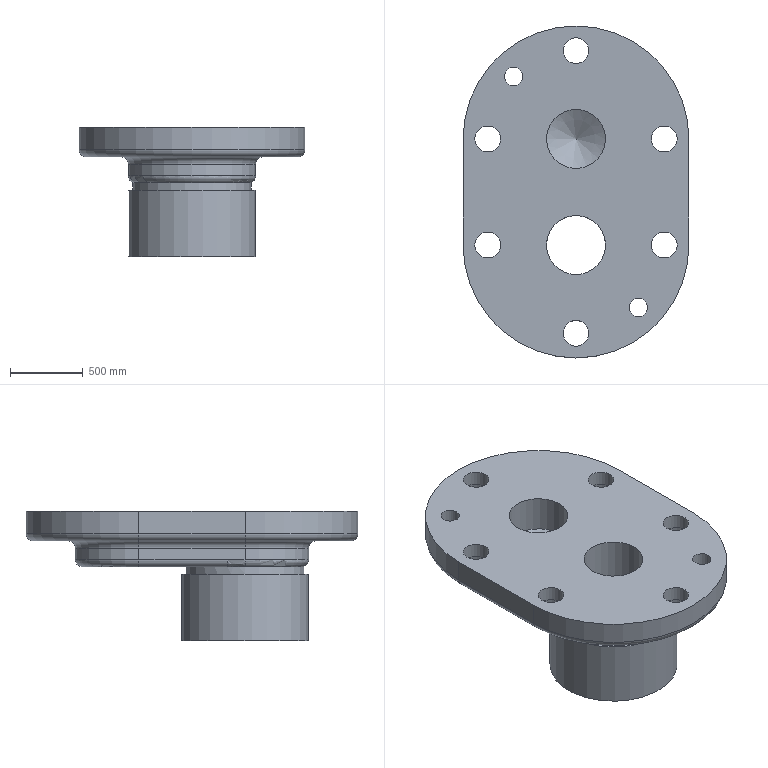Component | NX | 7YOUDUANGAI | 1 solid | 54 faces | volume 923047954 mm3 | cylinder 29 | plane 15 | torus 6 | cone 2 | spline 2 | commonest cylinder face diameters 177.8 x6 101.6 x6 228.6 x6 876.3 x3 1555.496 x2 127 x2 406.4 x2 812.8 x1